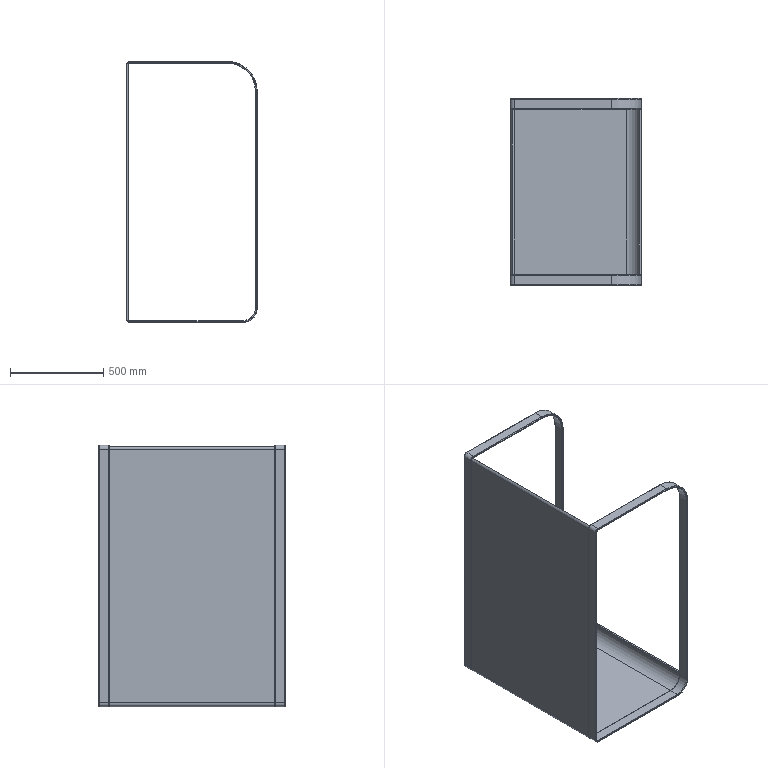Component | NX | HOUSING | 1 solid | 123 faces | volume 23288674 mm3 | cylinder 56 | plane 35 | torus 32 | commonest cylinder face diameters 6 x32 40 x6 20 x5 140 x3 160 x3 320 x2 300 x2 100 x2